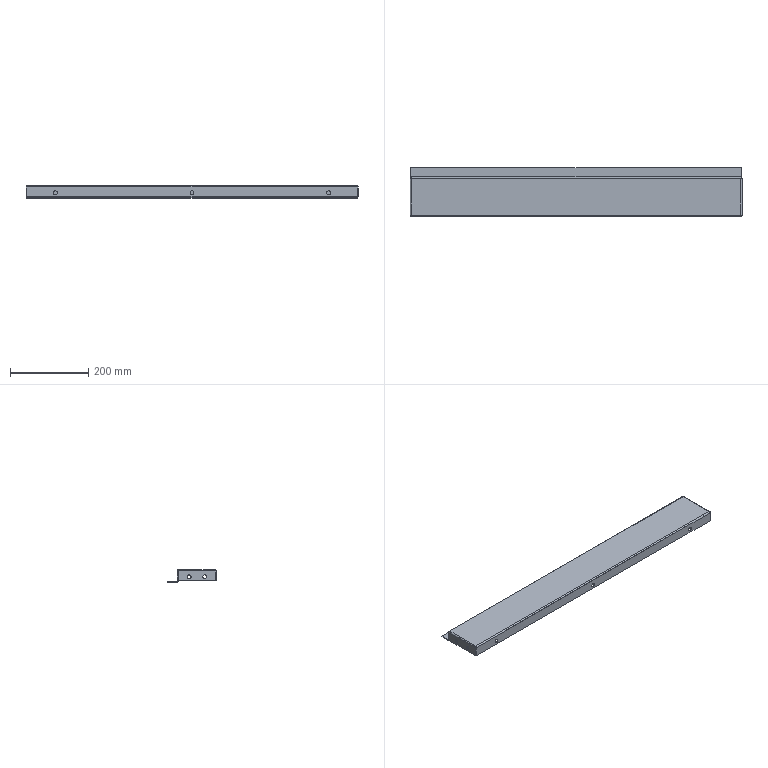Component | SolidWorks | 25BaseFrontSidePlateII-1 | 1 solid | 60 faces | volume 311111 mm3 | plane 28 | cylinder 24 | spline 8 | commonest cylinder face diameters 10 x14 2 x5 6 x5